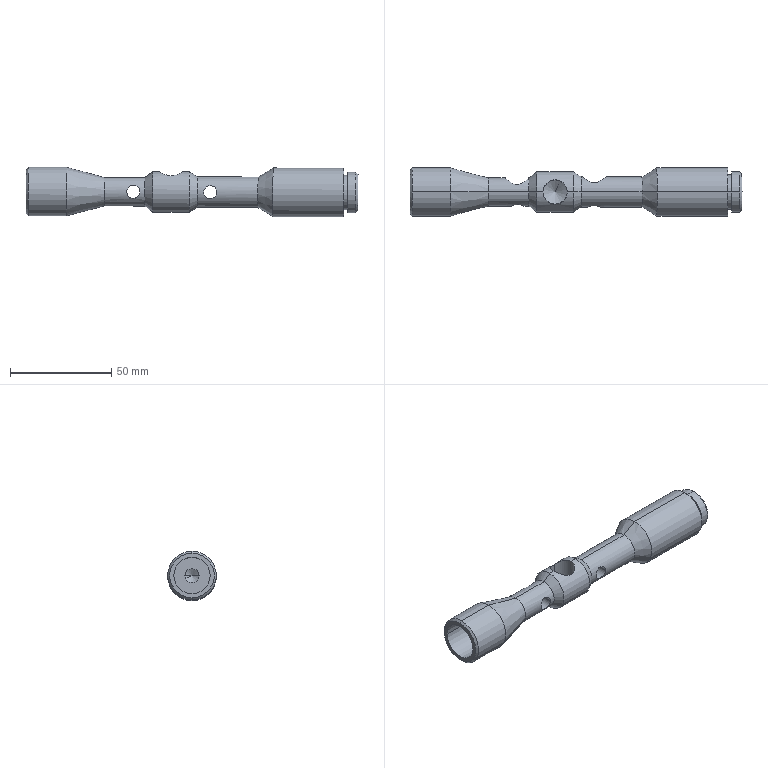Component | SolidWorks | Scope-1 | 1 solid | 59 faces | box 164.06 x 24 x 24.49 mm | volume 35414 mm3 | cylinder 32 | cone 18 | plane 9 | commonest cylinder face diameters 12 x6 6.5 x4 14 x4 24 x4 20 x4 18 x2 7 x2 10 x2
build123d program:
from build123d import *

# Parameters (mm, degrees)
CYLINDRICAL_COUNTERSUNK_HOLE_FOR_M6_HEX_D           = 10
CYLINDRICAL_COUNTERSUNK_HOLE_FOR_M6_HEX_DEPTH       = 50
CYLINDRICAL_COUNTERSUNK_HOLE_FOR_M6_HEX_CBORE_D     = 14
CYLINDRICAL_COUNTERSUNK_HOLE_FOR_M6_HEX_CBORE_DEPTH = 20
CYLINDRICAL_COUNTERSUNK_HOLE_FOR_M6_HEX_TIP         = 3.004
SKETCH17_R                                          = 6
CUT_EXTRUDE1_DEPTH                                  = 4
SKETCH18_R                                          = 3.25
CUT_EXTRUDE2_DEPTH                                  = 17
SKETCH19_R                                          = 6
CUT_EXTRUDE3_DEPTH                                  = 5
SKETCH20_R                                          = 3.25
CUT_EXTRUDE4_DEPTH                                  = 19
M12_TAPPED_HOLE2_D                                  = 12
M12_TAPPED_HOLE2_DEPTH                              = 16
M12_TAPPED_HOLE2_TIP                                = 3.605
CHAMFER1_SIZE                                       = 1


with BuildPart() as part:
    # Sketch1 → Revolve1 (revolve)
    with BuildSketch(Plane.XY, mode=Mode.PRIVATE) as revolve1_sk:
        Polygon((0, 0), (0, 10), (5, 10), (5, 8.5), (7, 8.5), (7, 12), (42, 12), (49.4, 7.5), (79.4, 7.5), (83.35, 10), (101.35, 10), (105.3, 7), (125.3, 7), (144, 12), (164, 12), (164, 0), align=None)
    revolve(revolve1_sk.sketch.rotate(Axis((-171.96, 0, 0), (1, 0, 0)), 180), axis=Axis((-171.96, 0, 0), (1, 0, 0)))

    # Cylindrical Countersunk Hole for M6 Hex
    with Locations(Plane(origin=(0, 0, 0), x_dir=(0, -1, 0), z_dir=(-1, 0, 0))):
        with Locations((0, 0)):
            CounterBoreHole(CYLINDRICAL_COUNTERSUNK_HOLE_FOR_M6_HEX_D / 2, CYLINDRICAL_COUNTERSUNK_HOLE_FOR_M6_HEX_CBORE_D / 2, CYLINDRICAL_COUNTERSUNK_HOLE_FOR_M6_HEX_CBORE_DEPTH, depth=CYLINDRICAL_COUNTERSUNK_HOLE_FOR_M6_HEX_DEPTH)
            with Locations((0, 0, -(CYLINDRICAL_COUNTERSUNK_HOLE_FOR_M6_HEX_DEPTH + CYLINDRICAL_COUNTERSUNK_HOLE_FOR_M6_HEX_TIP / 2))):  # 118° drill point
                Cone(0, CYLINDRICAL_COUNTERSUNK_HOLE_FOR_M6_HEX_D / 2, CYLINDRICAL_COUNTERSUNK_HOLE_FOR_M6_HEX_TIP, mode=Mode.SUBTRACT)

    # Sketch10 → Cylindrical Countersunk Hole for M6  2 (revolve, cut)
    with BuildSketch(Plane(origin=(164, 0, 0), x_dir=(0, 0, -1), z_dir=(0, 1, 0))):
        Polygon((0, 0), (0, 47.103), (3.5, 45), (3.5, 20), (9, 20), (9, 0), align=None)
    revolve(axis=Axis((170.35, 0, 0), (-1, 0, 0)), mode=Mode.SUBTRACT)

    # Sketch17 → Cut-Extrude1 (cut)
    with BuildSketch(Plane.XY.offset(7.5)):
        with Locations((73, 0)):
            Circle(SKETCH17_R)
    extrude(amount=-CUT_EXTRUDE1_DEPTH, mode=Mode.SUBTRACT)

    # Sketch18 → Cut-Extrude2 (cut)
    with BuildSketch(Plane.XY.offset(3.5)):
        with Locations((73, 0)):
            Circle(SKETCH18_R)
    extrude(amount=-CUT_EXTRUDE2_DEPTH, mode=Mode.SUBTRACT)

    # Sketch19 → Cut-Extrude3 (cut)
    with BuildSketch(Plane.XY.offset(7)):
        with Locations((111, 0)):
            Circle(SKETCH19_R)
    extrude(amount=-CUT_EXTRUDE3_DEPTH, mode=Mode.SUBTRACT)

    # Sketch20 → Cut-Extrude4 (cut)
    with BuildSketch(Plane.XY.offset(2)):
        with Locations((111, 0)):
            Circle(SKETCH20_R)
    extrude(amount=-CUT_EXTRUDE4_DEPTH, mode=Mode.SUBTRACT)

    # M12 Tapped Hole2
    with Locations(Plane(origin=(0, 10, 0), x_dir=(1, 0, 0), z_dir=(0, 1, 0))):
        with Locations((92.35, 0)):
            Hole(M12_TAPPED_HOLE2_D / 2, depth=M12_TAPPED_HOLE2_DEPTH)
            with Locations((0, 0, -(M12_TAPPED_HOLE2_DEPTH + M12_TAPPED_HOLE2_TIP / 2))):  # 118° drill point
                Cone(0, M12_TAPPED_HOLE2_D / 2, M12_TAPPED_HOLE2_TIP, mode=Mode.SUBTRACT)

    # Chamfer1
    chamfer1_edges = [part.edges().sort_by_distance(p)[0] for p in [
        (164, 12, 0),
        (0, 10, 0),
    ]]
    chamfer(chamfer1_edges, length=CHAMFER1_SIZE)


solid = part.part

# Placed as in the assembly
solid = solid.moved(Location((76.932, 70.983, 1008.651), (-90.001, 0, -179.82)))